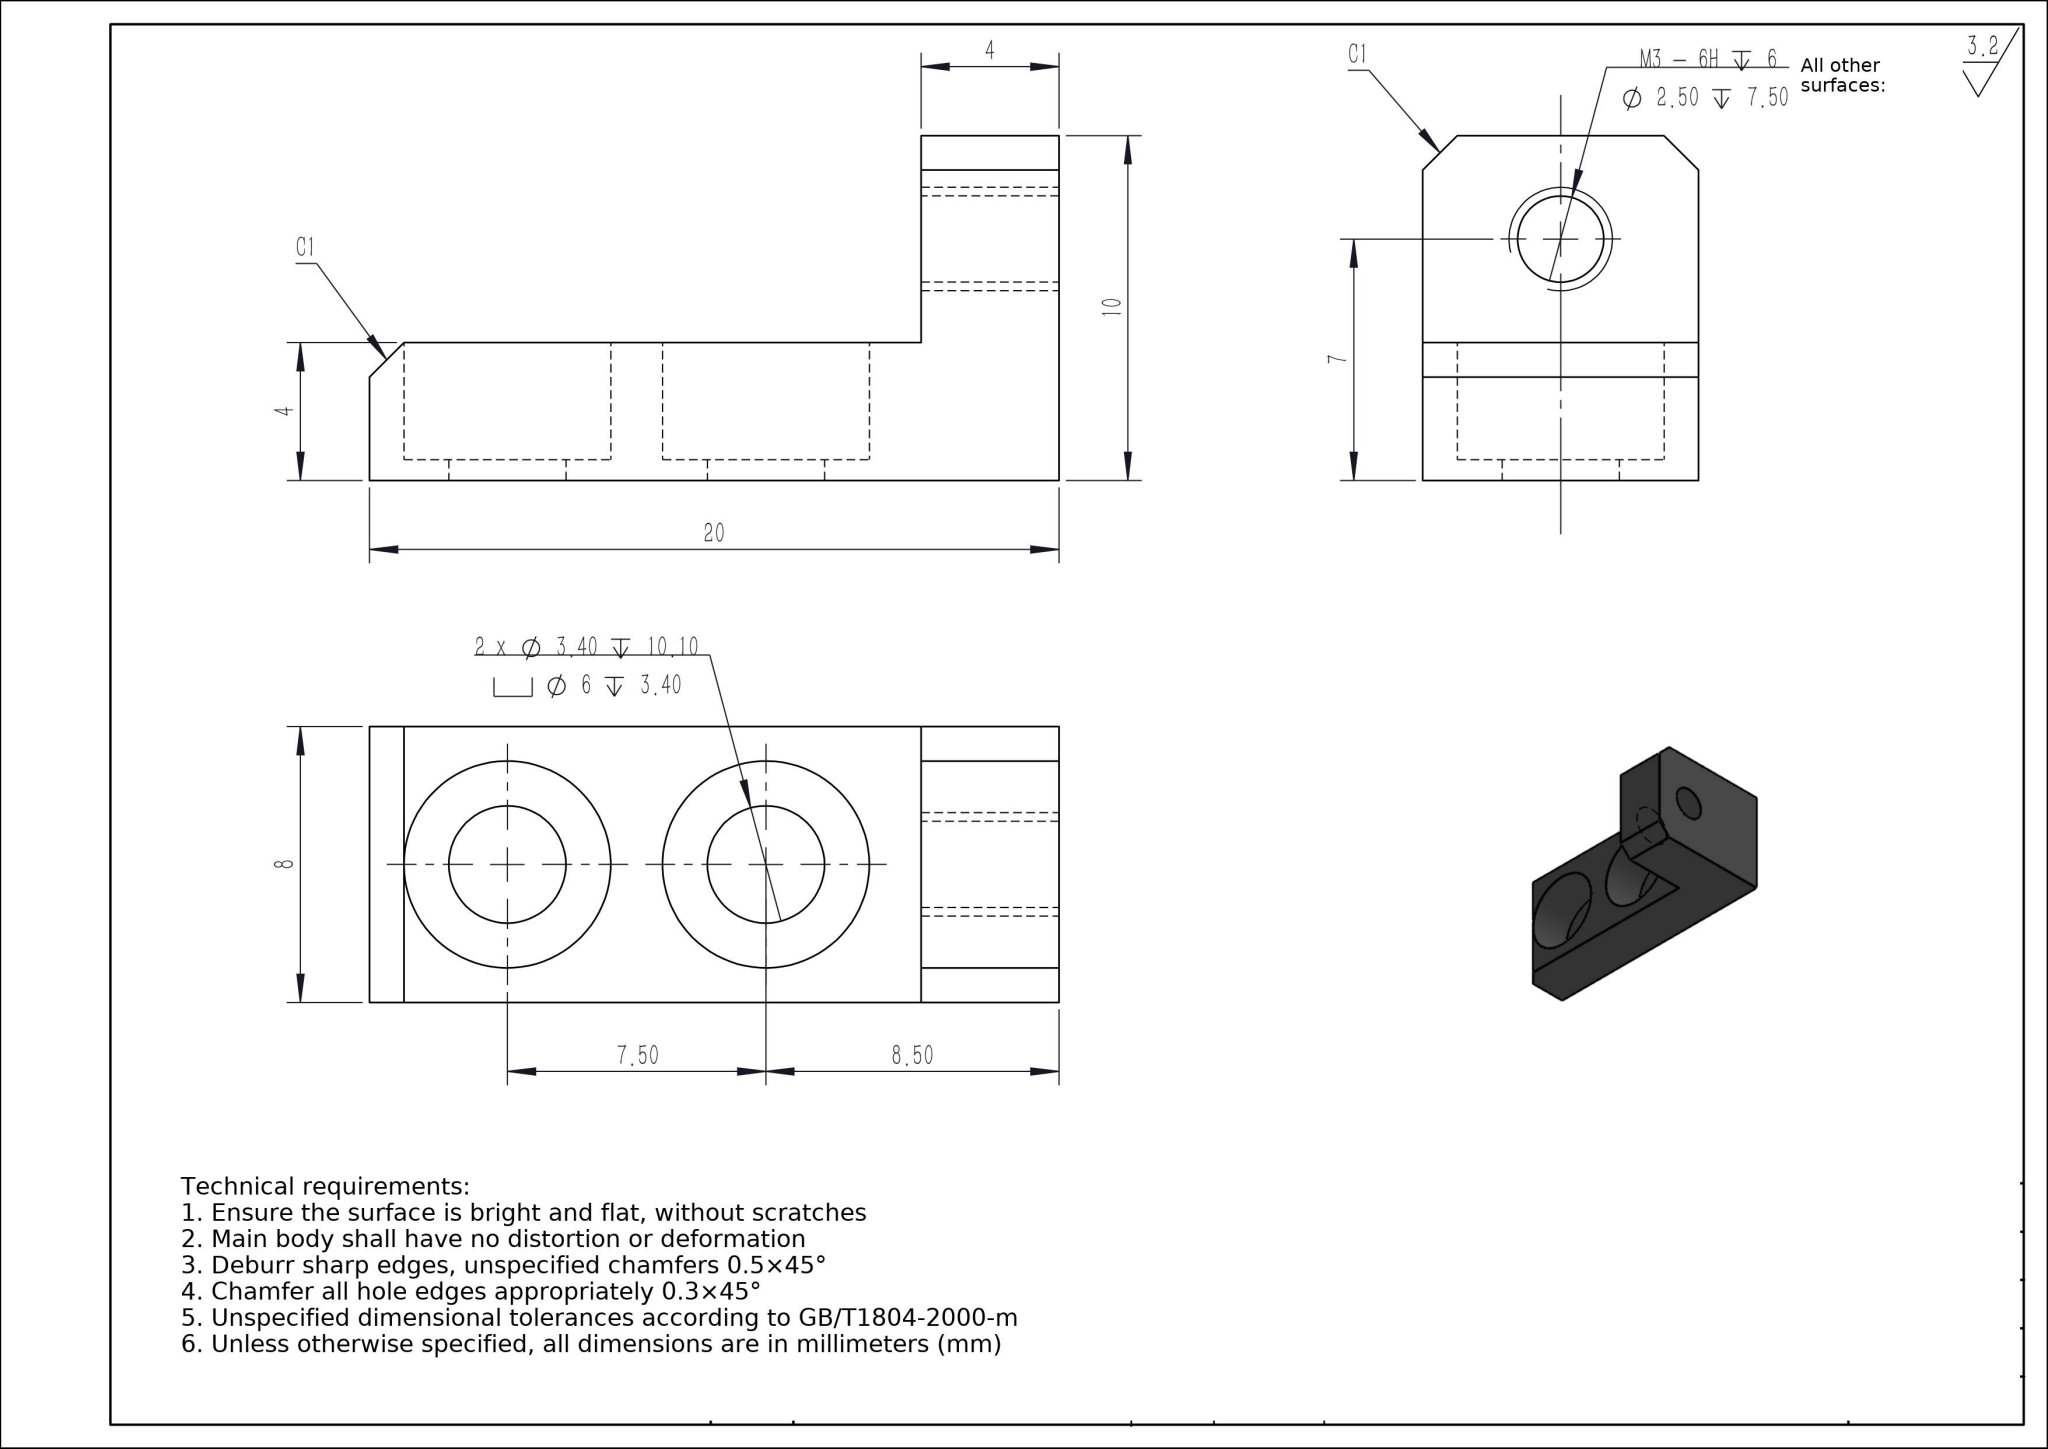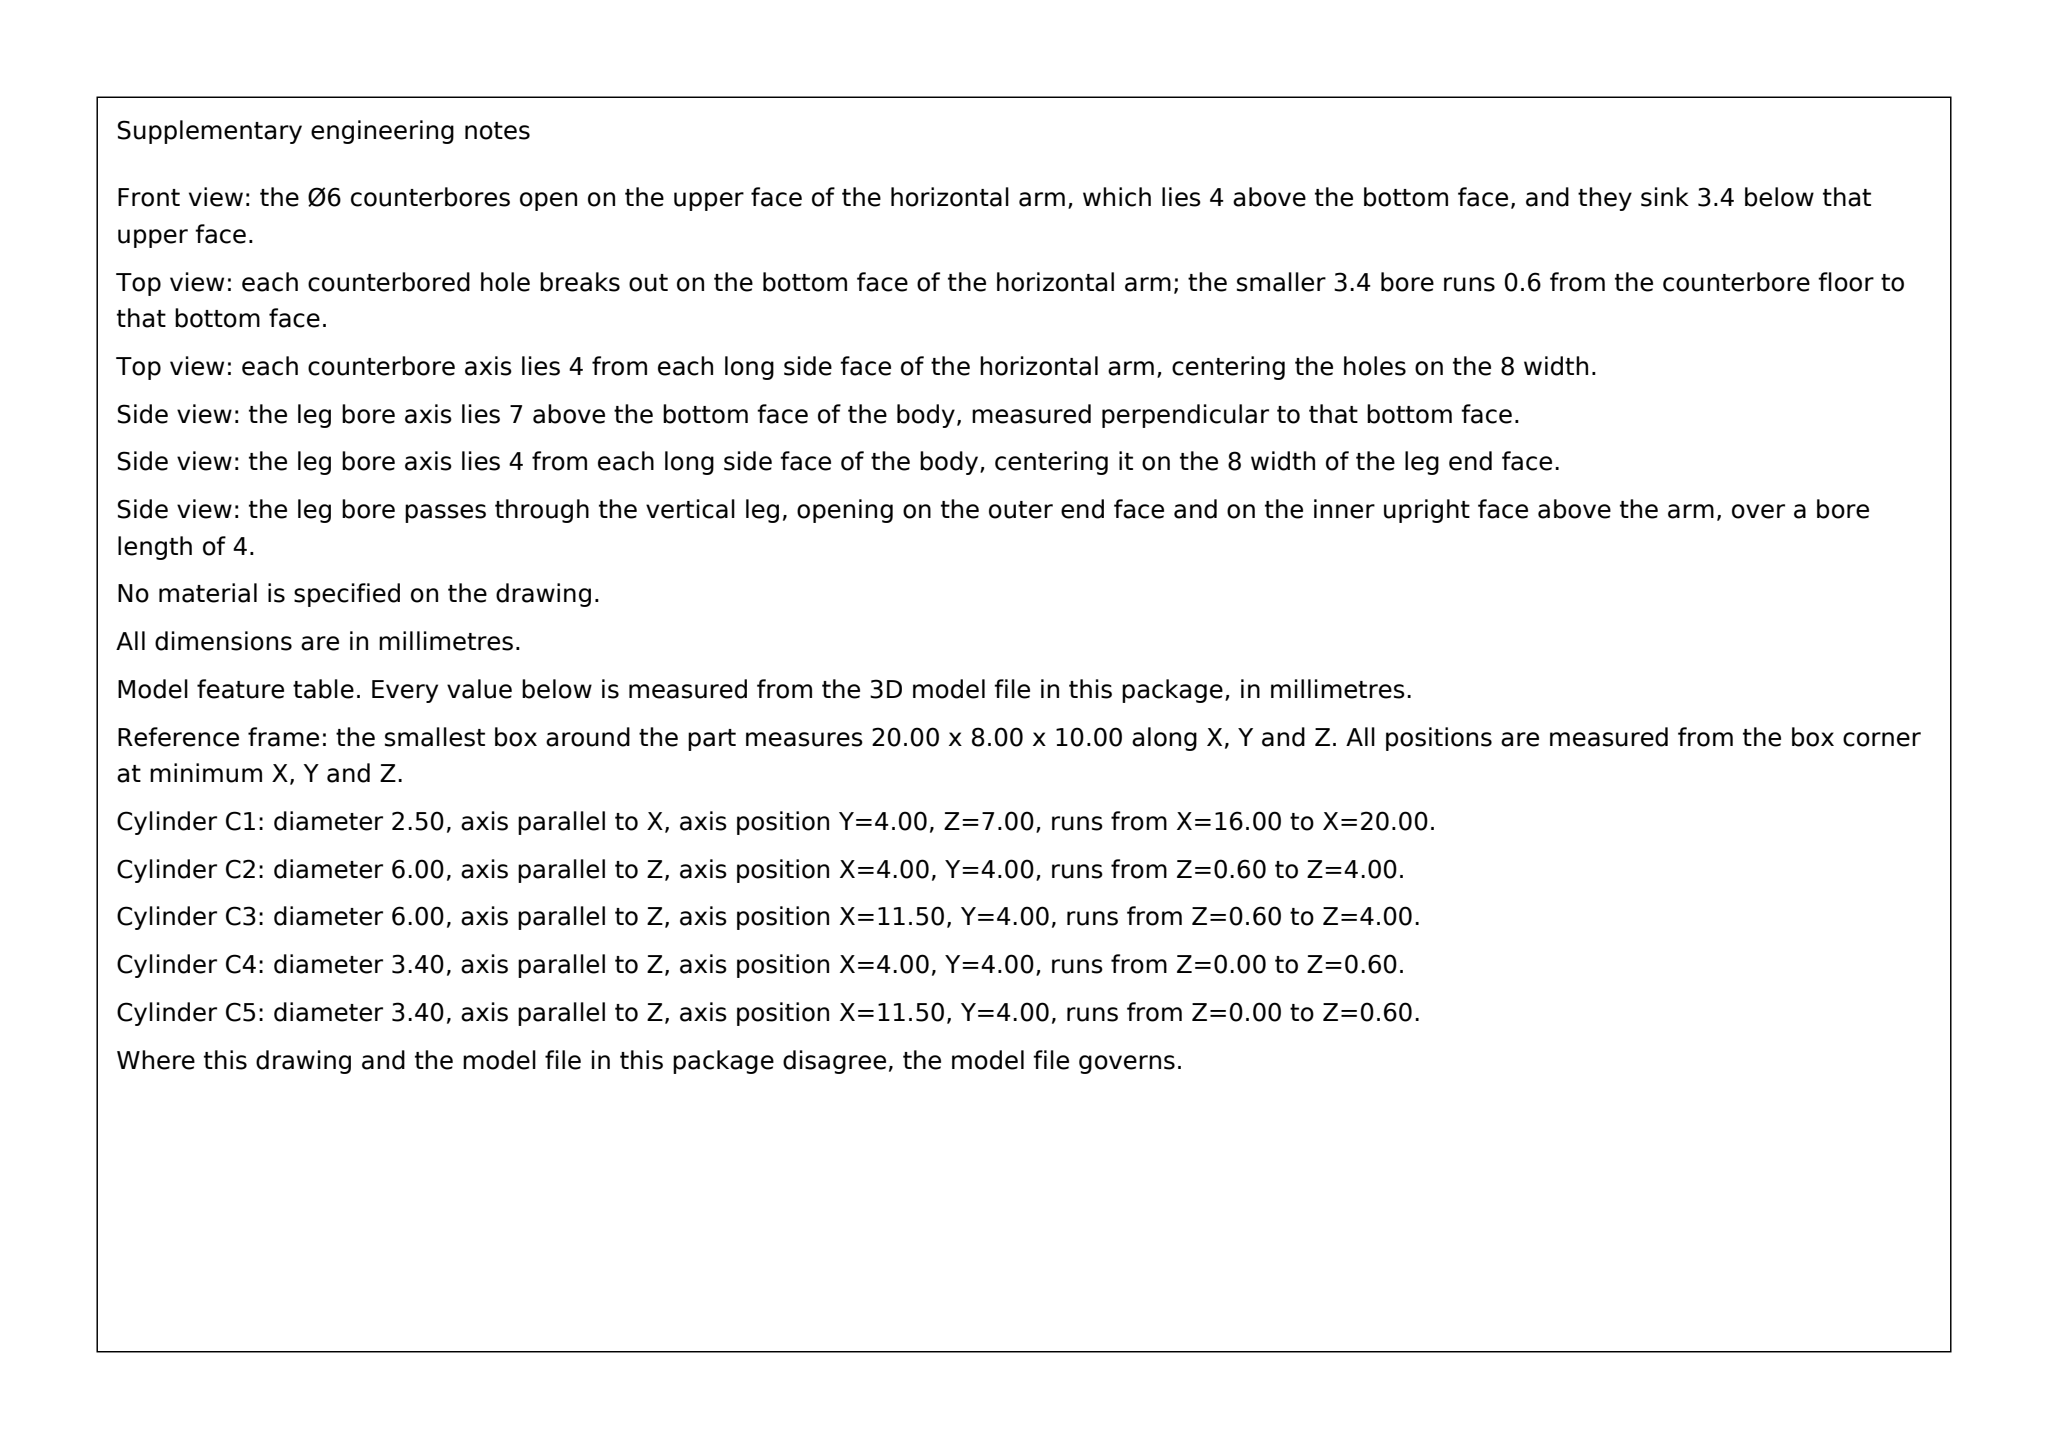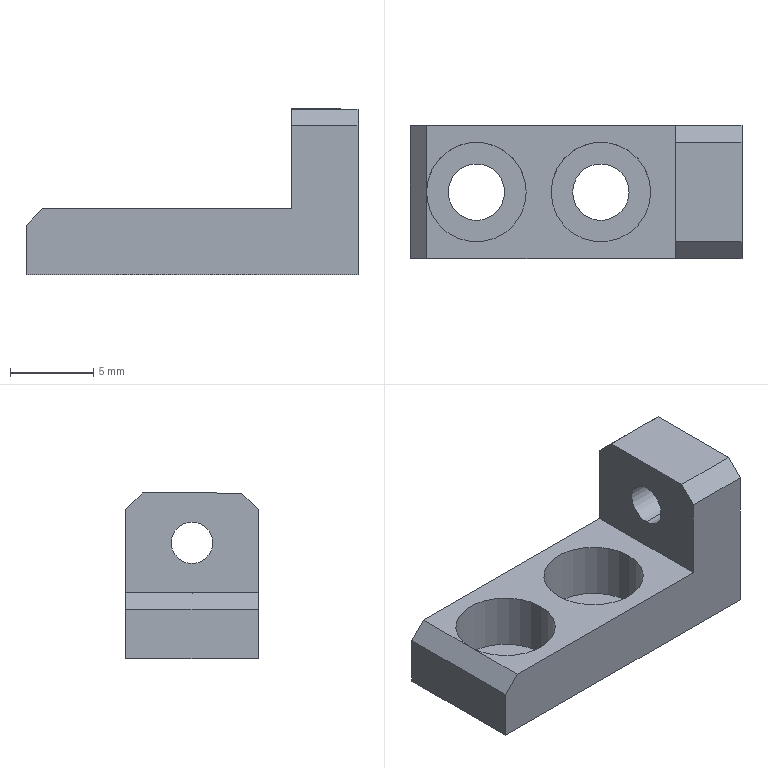Part | SolidWorks | mm | 1 solid | 23 faces | box 20 x 8 x 10 mm | volume 601 mm3 | plane 13 | cylinder 10 | commonest cylinder face diameters 6 x4 3.4 x4 2.5 x2
Drawing notes:
UPRIGHT TOP CORNERS: 2 x C1 (1 x 45 DEG) CHAMFER | from the solid: inclined_planes: two 45 deg faces, size [4,1,1] at bbox_from [16,0,9] and [16,7,9] -> 1x1 chamfer each side of 4 wide upright top edges
STEP:
#1=CARTESIAN_POINT('',(10.,-0.,5.75));
#2=VERTEX_POINT('',#1);
#3=CARTESIAN_POINT('',(10.,-0.,8.25));
#4=VERTEX_POINT('',#3);
#5=CARTESIAN_POINT('',(10.,-0.,7.));
#6=DIRECTION('',(-1.,0.,0.));
#7=DIRECTION('',(0.,0.,1.));
#8=AXIS2_PLACEMENT_3D('',#5,#6,#7);
#9=CIRCLE('',#8,1.25);
#10=EDGE_CURVE('',#2,#4,#9,.T.);
#11=ORIENTED_EDGE('',*,*,#10,.F.);
#12=CARTESIAN_POINT('',(6.,-0.,5.75));
#13=VERTEX_POINT('',#12);
#14=CARTESIAN_POINT('',(6.,-0.,5.75));
#15=DIRECTION('',(-1.,0.,0.));
#16=VECTOR('',#15,1000.);
#17=LINE('',#14,#16);
#18=EDGE_CURVE('',#2,#13,#17,.T.);
#19=ORIENTED_EDGE('',*,*,#18,.T.);
#20=CARTESIAN_POINT('',(6.,-0.,8.25));
#21=VERTEX_POINT('',#20);
#22=CARTESIAN_POINT('',(6.,-0.,7.));
#23=DIRECTION('',(-1.,0.,0.));
#24=DIRECTION('',(0.,0.,1.));
#25=AXIS2_PLACEMENT_3D('',#22,#23,#24);
#26=CIRCLE('',#25,1.25);
#27=EDGE_CURVE('',#13,#21,#26,.T.);
#28=ORIENTED_EDGE('',*,*,#27,.T.);
#29=CARTESIAN_POINT('',(6.,-0.,8.25));
#30=DIRECTION('',(-1.,0.,0.));
#31=VECTOR('',#30,1000.);
#32=LINE('',#29,#31);
#33=EDGE_CURVE('',#4,#21,#32,.T.);
#34=ORIENTED_EDGE('',*,*,#33,.F.);
#35=EDGE_LOOP('',(#11,#19,#28,#34));
#36=FACE_OUTER_BOUND('',#35,.T.);
#37=CARTESIAN_POINT('',(6.,-0.,7.));
#38=DIRECTION('',(-1.,0.,0.));
#39=DIRECTION('',(0.,0.,1.));
#40=AXIS2_PLACEMENT_3D('',#37,#38,#39);
#41=CYLINDRICAL_SURFACE('',#40,1.25);
#42=ADVANCED_FACE('',(#36),#41,.F.);
#43=CARTESIAN_POINT('',(-9.,0.,0.6));
#44=VERTEX_POINT('',#43);
#45=CARTESIAN_POINT('',(-3.,0.,0.6));
#46=VERTEX_POINT('',#45);
#47=CARTESIAN_POINT('',(-6.,0.,0.6));
#48=DIRECTION('',(0.,0.,1.));
#49=DIRECTION('',(1.,0.,0.));
#50=AXIS2_PLACEMENT_3D('',#47,#48,#49);
#51=CIRCLE('',#50,3.);
#52=EDGE_CURVE('',#44,#46,#51,.T.);
#53=ORIENTED_EDGE('',*,*,#52,.F.);
#54=CARTESIAN_POINT('',(-9.,0.,4.));
#55=VERTEX_POINT('',#54);
#56=CARTESIAN_POINT('',(-9.,0.,4.));
#57=DIRECTION('',(0.,0.,1.));
#58=VECTOR('',#57,1000.);
#59=LINE('',#56,#58);
#60=EDGE_CURVE('',#44,#55,#59,.T.);
#61=ORIENTED_EDGE('',*,*,#60,.T.);
#62=CARTESIAN_POINT('',(-3.,0.,4.));
#63=VERTEX_POINT('',#62);
#64=CARTESIAN_POINT('',(-6.,0.,4.));
#65=DIRECTION('',(0.,0.,1.));
#66=DIRECTION('',(1.,0.,0.));
#67=AXIS2_PLACEMENT_3D('',#64,#65,#66);
#68=CIRCLE('',#67,3.);
#69=EDGE_CURVE('',#55,#63,#68,.T.);
#70=ORIENTED_EDGE('',*,*,#69,.T.);
#71=CARTESIAN_POINT('',(-3.,0.,4.));
#72=DIRECTION('',(0.,0.,1.));
#73=VECTOR('',#72,1000.);
#74=LINE('',#71,#73);
#75=EDGE_CURVE('',#46,#63,#74,.T.);
#76=ORIENTED_EDGE('',*,*,#75,.F.);
#77=EDGE_LOOP('',(#53,#61,#70,#76));
#78=FACE_OUTER_BOUND('',#77,.T.);
#79=CARTESIAN_POINT('',(-6.,0.,4.));
#80=DIRECTION('',(0.,0.,1.));
#81=DIRECTION('',(1.,0.,0.));
#82=AXIS2_PLACEMENT_3D('',#79,#80,#81);
#83=CYLINDRICAL_SURFACE('',#82,3.);
#84=ADVANCED_FACE('',(#78),#83,.F.);
#85=CARTESIAN_POINT('',(-7.7,0.,0.));
#86=VERTEX_POINT('',#85);
#87=CARTESIAN_POINT('',(-4.3,0.,0.));
#88=VERTEX_POINT('',#87);
#89=CARTESIAN_POINT('',(-6.,0.,0.));
#90=DIRECTION('',(0.,0.,1.));
#91=DIRECTION('',(1.,0.,0.));
#92=AXIS2_PLACEMENT_3D('',#89,#90,#91);
#93=CIRCLE('',#92,1.7);
#94=EDGE_CURVE('',#86,#88,#93,.T.);
#95=ORIENTED_EDGE('',*,*,#94,.F.);
#96=CARTESIAN_POINT('',(-7.7,0.,0.6));
#97=VERTEX_POINT('',#96);
#98=CARTESIAN_POINT('',(-7.7,0.,4.));
#99=DIRECTION('',(0.,0.,1.));
#100=VECTOR('',#99,1000.);
#101=LINE('',#98,#100);
#102=EDGE_CURVE('',#86,#97,#101,.T.);
#103=ORIENTED_EDGE('',*,*,#102,.T.);
#104=CARTESIAN_POINT('',(-4.3,0.,0.6));
#105=VERTEX_POINT('',#104);
#106=CARTESIAN_POINT('',(-6.,0.,0.6));
#107=DIRECTION('',(0.,0.,1.));
#108=DIRECTION('',(1.,0.,0.));
#109=AXIS2_PLACEMENT_3D('',#106,#107,#108);
#110=CIRCLE('',#109,1.7);
#111=EDGE_CURVE('',#97,#105,#110,.T.);
#112=ORIENTED_EDGE('',*,*,#111,.T.);
#113=CARTESIAN_POINT('',(-4.3,0.,4.));
#114=DIRECTION('',(0.,0.,1.));
#115=VECTOR('',#114,1000.);
#116=LINE('',#113,#115);
#117=EDGE_CURVE('',#88,#105,#116,.T.);
#118=ORIENTED_EDGE('',*,*,#117,.F.);
#119=EDGE_LOOP('',(#95,#103,#112,#118));
#120=FACE_OUTER_BOUND('',#119,.T.);
#121=CARTESIAN_POINT('',(-6.,0.,4.));
#122=DIRECTION('',(0.,0.,1.));
#123=DIRECTION('',(1.,0.,0.));
#124=AXIS2_PLACEMENT_3D('',#121,#122,#123);
#125=CYLINDRICAL_SURFACE('',#124,1.7);
#126=ADVANCED_FACE('',(#120),#125,.F.);
#127=CARTESIAN_POINT('',(-1.5,0.,0.6));
#128=VERTEX_POINT('',#127);
#129=CARTESIAN_POINT('',(4.5,0.,0.6));
#130=VERTEX_POINT('',#129);
#131=CARTESIAN_POINT('',(1.5,0.,0.6));
#132=DIRECTION('',(0.,0.,1.));
#133=DIRECTION('',(1.,0.,0.));
#134=AXIS2_PLACEMENT_3D('',#131,#132,#133);
#135=CIRCLE('',#134,3.);
#136=EDGE_CURVE('',#128,#130,#135,.T.);
#137=ORIENTED_EDGE('',*,*,#136,.F.);
#138=CARTESIAN_POINT('',(-1.5,0.,4.));
#139=VERTEX_POINT('',#138);
#140=CARTESIAN_POINT('',(-1.5,0.,4.));
#141=DIRECTION('',(0.,0.,1.));
#142=VECTOR('',#141,1000.);
#143=LINE('',#140,#142);
#144=EDGE_CURVE('',#128,#139,#143,.T.);
#145=ORIENTED_EDGE('',*,*,#144,.T.);
#146=CARTESIAN_POINT('',(4.5,0.,4.));
#147=VERTEX_POINT('',#146);
#148=CARTESIAN_POINT('',(1.5,0.,4.));
#149=DIRECTION('',(0.,0.,1.));
#150=DIRECTION('',(1.,0.,0.));
#151=AXIS2_PLACEMENT_3D('',#148,#149,#150);
#152=CIRCLE('',#151,3.);
#153=EDGE_CURVE('',#139,#147,#152,.T.);
#154=ORIENTED_EDGE('',*,*,#153,.T.);
#155=CARTESIAN_POINT('',(4.5,0.,4.));
#156=DIRECTION('',(0.,0.,1.));
#157=VECTOR('',#156,1000.);
#158=LINE('',#155,#157);
#159=EDGE_CURVE('',#130,#147,#158,.T.);
#160=ORIENTED_EDGE('',*,*,#159,.F.);
#161=EDGE_LOOP('',(#137,#145,#154,#160));
#162=FACE_OUTER_BOUND('',#161,.T.);
#163=CARTESIAN_POINT('',(1.5,0.,4.));
#164=DIRECTION('',(0.,0.,1.));
#165=DIRECTION('',(1.,0.,0.));
#166=AXIS2_PLACEMENT_3D('',#163,#164,#165);
#167=CYLINDRICAL_SURFACE('',#166,3.);
#168=ADVANCED_FACE('',(#162),#167,.F.);
#169=CARTESIAN_POINT('',(-0.2,0.,0.));
#170=VERTEX_POINT('',#169);
#171=CARTESIAN_POINT('',(3.2,0.,0.));
#172=VERTEX_POINT('',#171);
#173=CARTESIAN_POINT('',(1.5,0.,0.));
#174=DIRECTION('',(0.,0.,1.));
#175=DIRECTION('',(1.,0.,0.));
#176=AXIS2_PLACEMENT_3D('',#173,#174,#175);
#177=CIRCLE('',#176,1.7);
#178=EDGE_CURVE('',#170,#172,#177,.T.);
#179=ORIENTED_EDGE('',*,*,#178,.F.);
#180=CARTESIAN_POINT('',(-0.2,0.,0.6));
#181=VERTEX_POINT('',#180);
#182=CARTESIAN_POINT('',(-0.2,0.,4.));
#183=DIRECTION('',(0.,0.,1.));
#184=VECTOR('',#183,1000.);
#185=LINE('',#182,#184);
#186=EDGE_CURVE('',#170,#181,#185,.T.);
#187=ORIENTED_EDGE('',*,*,#186,.T.);
#188=CARTESIAN_POINT('',(3.2,0.,0.6));
#189=VERTEX_POINT('',#188);
#190=CARTESIAN_POINT('',(1.5,0.,0.6));
#191=DIRECTION('',(0.,0.,1.));
#192=DIRECTION('',(1.,0.,0.));
#193=AXIS2_PLACEMENT_3D('',#190,#191,#192);
#194=CIRCLE('',#193,1.7);
#195=EDGE_CURVE('',#181,#189,#194,.T.);
#196=ORIENTED_EDGE('',*,*,#195,.T.);
#197=CARTESIAN_POINT('',(3.2,0.,4.));
#198=DIRECTION('',(0.,0.,1.));
#199=VECTOR('',#198,1000.);
#200=LINE('',#197,#199);
#201=EDGE_CURVE('',#172,#189,#200,.T.);
#202=ORIENTED_EDGE('',*,*,#201,.F.);
#203=EDGE_LOOP('',(#179,#187,#196,#202));
#204=FACE_OUTER_BOUND('',#203,.T.);
#205=CARTESIAN_POINT('',(1.5,0.,4.));
#206=DIRECTION('',(0.,0.,1.));
#207=DIRECTION('',(1.,0.,0.));
#208=AXIS2_PLACEMENT_3D('',#205,#206,#207);
#209=CYLINDRICAL_SURFACE('',#208,1.7);
#210=ADVANCED_FACE('',(#204),#209,.F.);
#211=CARTESIAN_POINT('',(-10.,-4.,3.));
#212=VERTEX_POINT('',#211);
#213=CARTESIAN_POINT('',(-10.,-4.,0.));
#214=VERTEX_POINT('',#213);
#215=CARTESIAN_POINT('',(-10.,-4.,4.));
#216=DIRECTION('',(0.,0.,-1.));
#217=VECTOR('',#216,1000.);
#218=LINE('',#215,#217);
#219=EDGE_CURVE('',#212,#214,#218,.T.);
#220=ORIENTED_EDGE('',*,*,#219,.F.);
#221=CARTESIAN_POINT('',(-10.,4.,3.));
#222=VERTEX_POINT('',#221);
#223=CARTESIAN_POINT('',(-10.,4.,3.));
#224=DIRECTION('',(0.,1.,0.));
#225=VECTOR('',#224,1000.);
#226=LINE('',#223,#225);
#227=EDGE_CURVE('',#212,#222,#226,.T.);
#228=ORIENTED_EDGE('',*,*,#227,.T.);
#229=CARTESIAN_POINT('',(-10.,4.,0.));
#230=VERTEX_POINT('',#229);
#231=CARTESIAN_POINT('',(-10.,4.,4.));
#232=DIRECTION('',(0.,0.,-1.));
#233=VECTOR('',#232,1000.);
#234=LINE('',#231,#233);
#235=EDGE_CURVE('',#222,#230,#234,.T.);
#236=ORIENTED_EDGE('',*,*,#235,.T.);
#237=CARTESIAN_POINT('',(-10.,-4.,0.));
#238=DIRECTION('',(0.,-1.,0.));
#239=VECTOR('',#238,1000.);
#240=LINE('',#237,#239);
#241=EDGE_CURVE('',#230,#214,#240,.T.);
#242=ORIENTED_EDGE('',*,*,#241,.T.);
#243=EDGE_LOOP('',(#220,#228,#236,#242));
#244=FACE_OUTER_BOUND('',#243,.T.);
#245=CARTESIAN_POINT('',(-10.,-4.,4.));
#246=DIRECTION('',(1.,0.,0.));
#247=DIRECTION('',(0.,0.,-1.));
#248=AXIS2_PLACEMENT_3D('',#245,#246,#247);
#249=PLANE('',#248);
#250=ADVANCED_FACE('',(#244),#249,.F.);
#251=CARTESIAN_POINT('',(10.,-4.,9.));
#252=VERTEX_POINT('',#251);
#253=CARTESIAN_POINT('',(10.,-4.,0.));
#254=VERTEX_POINT('',#253);
#255=CARTESIAN_POINT('',(10.,-4.,4.));
#256=DIRECTION('',(0.,0.,-1.));
#257=VECTOR('',#256,1000.);
#258=LINE('',#255,#257);
#259=EDGE_CURVE('',#252,#254,#258,.T.);
#260=ORIENTED_EDGE('',*,*,#259,.F.);
#261=CARTESIAN_POINT('',(6.,-4.,9.));
#262=VERTEX_POINT('',#261);
#263=CARTESIAN_POINT('',(6.,-4.,9.));
#264=DIRECTION('',(-1.,-0.,0.));
#265=VECTOR('',#264,1000.);
#266=LINE('',#263,#265);
#267=EDGE_CURVE('',#252,#262,#266,.T.);
#268=ORIENTED_EDGE('',*,*,#267,.T.);
#269=CARTESIAN_POINT('',(6.,-4.,4.));
#270=VERTEX_POINT('',#269);
#271=CARTESIAN_POINT('',(6.,-4.,10.));
#272=DIRECTION('',(0.,0.,-1.));
#273=VECTOR('',#272,1000.);
#274=LINE('',#271,#273);
#275=EDGE_CURVE('',#262,#270,#274,.T.);
#276=ORIENTED_EDGE('',*,*,#275,.T.);
#277=CARTESIAN_POINT('',(-9.,-4.,4.));
#278=VERTEX_POINT('',#277);
#279=CARTESIAN_POINT('',(10.,-4.,4.));
#280=DIRECTION('',(1.,0.,0.));
#281=VECTOR('',#280,1000.);
#282=LINE('',#279,#281);
#283=EDGE_CURVE('',#278,#270,#282,.T.);
#284=ORIENTED_EDGE('',*,*,#283,.F.);
#285=CARTESIAN_POINT('',(-9.,-4.,4.));
#286=DIRECTION('',(-0.7071,-0.,-0.7071));
#287=VECTOR('',#286,1000.);
#288=LINE('',#285,#287);
#289=EDGE_CURVE('',#278,#212,#288,.T.);
#290=ORIENTED_EDGE('',*,*,#289,.T.);
#291=ORIENTED_EDGE('',*,*,#219,.T.);
#292=CARTESIAN_POINT('',(10.,-4.,0.));
#293=DIRECTION('',(1.,0.,0.));
#294=VECTOR('',#293,1000.);
#295=LINE('',#292,#294);
#296=EDGE_CURVE('',#214,#254,#295,.T.);
#297=ORIENTED_EDGE('',*,*,#296,.T.);
#298=EDGE_LOOP('',(#260,#268,#276,#284,#290,#291,#297));
#299=FACE_OUTER_BOUND('',#298,.T.);
#300=CARTESIAN_POINT('',(10.,-4.,4.));
#301=DIRECTION('',(-0.,1.,0.));
#302=DIRECTION('',(-1.,-0.,0.));
#303=AXIS2_PLACEMENT_3D('',#300,#301,#302);
#304=PLANE('',#303);
#305=ADVANCED_FACE('',(#299),#304,.F.);
#306=CARTESIAN_POINT('',(10.,-0.,7.));
#307=DIRECTION('',(-1.,0.,0.));
#308=DIRECTION('',(0.,0.,1.));
#309=AXIS2_PLACEMENT_3D('',#306,#307,#308);
#310=CIRCLE('',#309,1.25);
#311=EDGE_CURVE('',#4,#2,#310,.T.);
#312=ORIENTED_EDGE('',*,*,#311,.T.);
#313=ORIENTED_EDGE('',*,*,#10,.T.);
#314=EDGE_LOOP('',(#312,#313));
#315=FACE_BOUND('',#314,.T.);
#316=CARTESIAN_POINT('',(10.,4.,9.));
#317=VERTEX_POINT('',#316);
#318=CARTESIAN_POINT('',(10.,4.,0.));
#319=VERTEX_POINT('',#318);
#320=CARTESIAN_POINT('',(10.,4.,4.));
#321=DIRECTION('',(0.,0.,-1.));
#322=VECTOR('',#321,1000.);
#323=LINE('',#320,#322);
#324=EDGE_CURVE('',#317,#319,#323,.T.);
#325=ORIENTED_EDGE('',*,*,#324,.F.);
#326=CARTESIAN_POINT('',(10.,3.,10.));
#327=VERTEX_POINT('',#326);
#328=CARTESIAN_POINT('',(10.,3.,10.));
#329=DIRECTION('',(0.,-0.7071,0.7071));
#330=VECTOR('',#329,1000.);
#331=LINE('',#328,#330);
#332=EDGE_CURVE('',#317,#327,#331,.T.);
#333=ORIENTED_EDGE('',*,*,#332,.T.);
#334=CARTESIAN_POINT('',(10.,-3.,10.));
#335=VERTEX_POINT('',#334);
#336=CARTESIAN_POINT('',(10.,-4.,10.));
#337=DIRECTION('',(0.,1.,0.));
#338=VECTOR('',#337,1000.);
#339=LINE('',#336,#338);
#340=EDGE_CURVE('',#335,#327,#339,.T.);
#341=ORIENTED_EDGE('',*,*,#340,.F.);
#342=CARTESIAN_POINT('',(10.,-3.,10.));
#343=DIRECTION('',(0.,-0.7071,-0.7071));
#344=VECTOR('',#343,1000.);
#345=LINE('',#342,#344);
#346=EDGE_CURVE('',#335,#252,#345,.T.);
#347=ORIENTED_EDGE('',*,*,#346,.T.);
#348=ORIENTED_EDGE('',*,*,#259,.T.);
#349=CARTESIAN_POINT('',(10.,-4.,0.));
#350=DIRECTION('',(0.,1.,0.));
#351=VECTOR('',#350,1000.);
#352=LINE('',#349,#351);
#353=EDGE_CURVE('',#254,#319,#352,.T.);
#354=ORIENTED_EDGE('',*,*,#353,.T.);
#355=EDGE_LOOP('',(#325,#333,#341,#347,#348,#354));
#356=FACE_OUTER_BOUND('',#355,.T.);
#357=CARTESIAN_POINT('',(10.,-4.,4.));
#358=DIRECTION('',(-1.,0.,0.));
#359=DIRECTION('',(0.,0.,1.));
#360=AXIS2_PLACEMENT_3D('',#357,#358,#359);
#361=PLANE('',#360);
#362=ADVANCED_FACE('',(#315,#356),#361,.F.);
#363=CARTESIAN_POINT('',(6.,4.,9.));
#364=VERTEX_POINT('',#363);
#365=CARTESIAN_POINT('',(6.,4.,4.));
#366=VERTEX_POINT('',#365);
#367=CARTESIAN_POINT('',(6.,4.,10.));
#368=DIRECTION('',(0.,0.,-1.));
#369=VECTOR('',#368,1000.);
#370=LINE('',#367,#369);
#371=EDGE_CURVE('',#364,#366,#370,.T.);
#372=ORIENTED_EDGE('',*,*,#371,.F.);
#373=CARTESIAN_POINT('',(10.,4.,9.));
#374=DIRECTION('',(1.,0.,0.));
#375=VECTOR('',#374,1000.);
#376=LINE('',#373,#375);
#377=EDGE_CURVE('',#364,#317,#376,.T.);
#378=ORIENTED_EDGE('',*,*,#377,.T.);
#379=ORIENTED_EDGE('',*,*,#324,.T.);
#380=CARTESIAN_POINT('',(10.,4.,0.));
#381=DIRECTION('',(-1.,-0.,0.));
#382=VECTOR('',#381,1000.);
#383=LINE('',#380,#382);
#384=EDGE_CURVE('',#319,#230,#383,.T.);
#385=ORIENTED_EDGE('',*,*,#384,.T.);
#386=ORIENTED_EDGE('',*,*,#235,.F.);
#387=CARTESIAN_POINT('',(-9.,4.,4.));
#388=VERTEX_POINT('',#387);
#389=CARTESIAN_POINT('',(-9.,4.,4.));
#390=DIRECTION('',(0.7071,0.,0.7071));
#391=VECTOR('',#390,1000.);
#392=LINE('',#389,#391);
#393=EDGE_CURVE('',#222,#388,#392,.T.);
#394=ORIENTED_EDGE('',*,*,#393,.T.);
#395=CARTESIAN_POINT('',(10.,4.,4.));
#396=DIRECTION('',(-1.,-0.,0.));
#397=VECTOR('',#396,1000.);
#398=LINE('',#395,#397);
#399=EDGE_CURVE('',#366,#388,#398,.T.);
#400=ORIENTED_EDGE('',*,*,#399,.F.);
#401=EDGE_LOOP('',(#372,#378,#379,#385,#386,#394,#400));
#402=FACE_OUTER_BOUND('',#401,.T.);
#403=CARTESIAN_POINT('',(10.,4.,4.));
#404=DIRECTION('',(0.,-1.,0.));
#405=DIRECTION('',(1.,0.,0.));
#406=AXIS2_PLACEMENT_3D('',#403,#404,#405);
#407=PLANE('',#406);
#408=ADVANCED_FACE('',(#402),#407,.F.);
#409=CARTESIAN_POINT('',(6.,-4.,4.));
#410=DIRECTION('',(0.,-1.,0.));
#411=VECTOR('',#410,1000.);
#412=LINE('',#409,#411);
#413=EDGE_CURVE('',#366,#270,#412,.T.);
#414=ORIENTED_EDGE('',*,*,#413,.F.);
#415=ORIENTED_EDGE('',*,*,#399,.T.);
#416=CARTESIAN_POINT('',(-9.,-4.,4.));
#417=DIRECTION('',(0.,-1.,0.));
#418=VECTOR('',#417,1000.);
#419=LINE('',#416,#418);
#420=EDGE_CURVE('',#388,#55,#419,.T.);
#421=ORIENTED_EDGE('',*,*,#420,.T.);
#422=CARTESIAN_POINT('',(-6.,0.,4.));
#423=DIRECTION('',(0.,0.,1.));
#424=DIRECTION('',(1.,0.,0.));
#425=AXIS2_PLACEMENT_3D('',#422,#423,#424);
#426=CIRCLE('',#425,3.);
#427=EDGE_CURVE('',#63,#55,#426,.T.);
#428=ORIENTED_EDGE('',*,*,#427,.F.);
#429=ORIENTED_EDGE('',*,*,#69,.F.);
#430=CARTESIAN_POINT('',(-9.,-4.,4.));
#431=DIRECTION('',(0.,-1.,0.));
#432=VECTOR('',#431,1000.);
#433=LINE('',#430,#432);
#434=EDGE_CURVE('',#55,#278,#433,.T.);
#435=ORIENTED_EDGE('',*,*,#434,.T.);
#436=ORIENTED_EDGE('',*,*,#283,.T.);
#437=EDGE_LOOP('',(#414,#415,#421,#428,#429,#435,#436));
#438=FACE_OUTER_BOUND('',#437,.T.);
#439=CARTESIAN_POINT('',(1.5,0.,4.));
#440=DIRECTION('',(0.,0.,1.));
#441=DIRECTION('',(1.,0.,0.));
#442=AXIS2_PLACEMENT_3D('',#439,#440,#441);
#443=CIRCLE('',#442,3.);
#444=EDGE_CURVE('',#147,#139,#443,.T.);
#445=ORIENTED_EDGE('',*,*,#444,.F.);
#446=ORIENTED_EDGE('',*,*,#153,.F.);
#447=EDGE_LOOP('',(#445,#446));
#448=FACE_BOUND('',#447,.T.);
#449=CARTESIAN_POINT('',(0.,0.,4.));
#450=DIRECTION('',(0.,0.,1.));
#451=DIRECTION('',(1.,0.,0.));
#452=AXIS2_PLACEMENT_3D('',#449,#450,#451);
#453=PLANE('',#452);
#454=ADVANCED_FACE('',(#438,#448),#453,.T.);
#455=CARTESIAN_POINT('',(-6.,0.,0.));
#456=DIRECTION('',(0.,0.,1.));
#457=DIRECTION('',(1.,0.,0.));
#458=AXIS2_PLACEMENT_3D('',#455,#456,#457);
#459=CIRCLE('',#458,1.7);
#460=EDGE_CURVE('',#88,#86,#459,.T.);
#461=ORIENTED_EDGE('',*,*,#460,.T.);
#462=ORIENTED_EDGE('',*,*,#94,.T.);
#463=EDGE_LOOP('',(#461,#462));
#464=FACE_BOUND('',#463,.T.);
#465=CARTESIAN_POINT('',(1.5,0.,0.));
#466=DIRECTION('',(0.,0.,1.));
#467=DIRECTION('',(1.,0.,0.));
#468=AXIS2_PLACEMENT_3D('',#465,#466,#467);
#469=CIRCLE('',#468,1.7);
#470=EDGE_CURVE('',#172,#170,#469,.T.);
#471=ORIENTED_EDGE('',*,*,#470,.T.);
#472=ORIENTED_EDGE('',*,*,#178,.T.);
#473=EDGE_LOOP('',(#471,#472));
#474=FACE_BOUND('',#473,.T.);
#475=ORIENTED_EDGE('',*,*,#241,.F.);
#476=ORIENTED_EDGE('',*,*,#384,.F.);
#477=ORIENTED_EDGE('',*,*,#353,.F.);
#478=ORIENTED_EDGE('',*,*,#296,.F.);
#479=EDGE_LOOP('',(#475,#476,#477,#478));
#480=FACE_OUTER_BOUND('',#479,.T.);
#481=CARTESIAN_POINT('',(0.,0.,0.));
#482=DIRECTION('',(0.,0.,1.));
#483=DIRECTION('',(1.,0.,0.));
#484=AXIS2_PLACEMENT_3D('',#481,#482,#483);
#485=PLANE('',#484);
#486=ADVANCED_FACE('',(#464,#474,#480),#485,.F.);
#487=ORIENTED_EDGE('',*,*,#186,.F.);
#488=ORIENTED_EDGE('',*,*,#470,.F.);
#489=ORIENTED_EDGE('',*,*,#201,.T.);
#490=CARTESIAN_POINT('',(1.5,0.,0.6));
#491=DIRECTION('',(0.,0.,1.));
#492=DIRECTION('',(1.,0.,0.));
#493=AXIS2_PLACEMENT_3D('',#490,#491,#492);
#494=CIRCLE('',#493,1.7);
#495=EDGE_CURVE('',#189,#181,#494,.T.);
#496=ORIENTED_EDGE('',*,*,#495,.T.);
#497=EDGE_LOOP('',(#487,#488,#489,#496));
#498=FACE_OUTER_BOUND('',#497,.T.);
#499=CARTESIAN_POINT('',(1.5,0.,4.));
#500=DIRECTION('',(0.,0.,1.));
#501=DIRECTION('',(1.,0.,0.));
#502=AXIS2_PLACEMENT_3D('',#499,#500,#501);
#503=CYLINDRICAL_SURFACE('',#502,1.7);
#504=ADVANCED_FACE('',(#498),#503,.F.);
#505=ORIENTED_EDGE('',*,*,#495,.F.);
#506=ORIENTED_EDGE('',*,*,#195,.F.);
#507=EDGE_LOOP('',(#505,#506));
#508=FACE_BOUND('',#507,.T.);
#509=CARTESIAN_POINT('',(1.5,0.,0.6));
#510=DIRECTION('',(0.,0.,1.));
#511=DIRECTION('',(1.,0.,0.));
#512=AXIS2_PLACEMENT_3D('',#509,#510,#511);
#513=CIRCLE('',#512,3.);
#514=EDGE_CURVE('',#130,#128,#513,.T.);
#515=ORIENTED_EDGE('',*,*,#514,.T.);
#516=ORIENTED_EDGE('',*,*,#136,.T.);
#517=EDGE_LOOP('',(#515,#516));
#518=FACE_OUTER_BOUND('',#517,.T.);
#519=CARTESIAN_POINT('',(3.2,0.,0.6));
#520=DIRECTION('',(0.,0.,-1.));
#521=DIRECTION('',(-1.,0.,0.));
#522=AXIS2_PLACEMENT_3D('',#519,#520,#521);
#523=PLANE('',#522);
#524=ADVANCED_FACE('',(#508,#518),#523,.F.);
#525=ORIENTED_EDGE('',*,*,#144,.F.);
#526=ORIENTED_EDGE('',*,*,#514,.F.);
#527=ORIENTED_EDGE('',*,*,#159,.T.);
#528=ORIENTED_EDGE('',*,*,#444,.T.);
#529=EDGE_LOOP('',(#525,#526,#527,#528));
#530=FACE_OUTER_BOUND('',#529,.T.);
#531=CARTESIAN_POINT('',(1.5,0.,4.));
#532=DIRECTION('',(0.,0.,1.));
#533=DIRECTION('',(1.,0.,0.));
#534=AXIS2_PLACEMENT_3D('',#531,#532,#533);
#535=CYLINDRICAL_SURFACE('',#534,3.);
#536=ADVANCED_FACE('',(#530),#535,.F.);
#537=ORIENTED_EDGE('',*,*,#102,.F.);
#538=ORIENTED_EDGE('',*,*,#460,.F.);
#539=ORIENTED_EDGE('',*,*,#117,.T.);
#540=CARTESIAN_POINT('',(-6.,0.,0.6));
#541=DIRECTION('',(0.,0.,1.));
#542=DIRECTION('',(1.,0.,0.));
#543=AXIS2_PLACEMENT_3D('',#540,#541,#542);
#544=CIRCLE('',#543,1.7);
#545=EDGE_CURVE('',#105,#97,#544,.T.);
#546=ORIENTED_EDGE('',*,*,#545,.T.);
#547=EDGE_LOOP('',(#537,#538,#539,#546));
#548=FACE_OUTER_BOUND('',#547,.T.);
#549=CARTESIAN_POINT('',(-6.,0.,4.));
#550=DIRECTION('',(0.,0.,1.));
#551=DIRECTION('',(1.,0.,0.));
#552=AXIS2_PLACEMENT_3D('',#549,#550,#551);
#553=CYLINDRICAL_SURFACE('',#552,1.7);
#554=ADVANCED_FACE('',(#548),#553,.F.);
#555=ORIENTED_EDGE('',*,*,#545,.F.);
#556=ORIENTED_EDGE('',*,*,#111,.F.);
#557=EDGE_LOOP('',(#555,#556));
#558=FACE_BOUND('',#557,.T.);
#559=CARTESIAN_POINT('',(-6.,0.,0.6));
#560=DIRECTION('',(0.,0.,1.));
#561=DIRECTION('',(1.,0.,0.));
#562=AXIS2_PLACEMENT_3D('',#559,#560,#561);
#563=CIRCLE('',#562,3.);
#564=EDGE_CURVE('',#46,#44,#563,.T.);
#565=ORIENTED_EDGE('',*,*,#564,.T.);
#566=ORIENTED_EDGE('',*,*,#52,.T.);
#567=EDGE_LOOP('',(#565,#566));
#568=FACE_OUTER_BOUND('',#567,.T.);
#569=CARTESIAN_POINT('',(-4.3,0.,0.6));
#570=DIRECTION('',(0.,0.,-1.));
#571=DIRECTION('',(-1.,0.,0.));
#572=AXIS2_PLACEMENT_3D('',#569,#570,#571);
#573=PLANE('',#572);
#574=ADVANCED_FACE('',(#558,#568),#573,.F.);
#575=ORIENTED_EDGE('',*,*,#60,.F.);
#576=ORIENTED_EDGE('',*,*,#564,.F.);
#577=ORIENTED_EDGE('',*,*,#75,.T.);
#578=ORIENTED_EDGE('',*,*,#427,.T.);
#579=EDGE_LOOP('',(#575,#576,#577,#578));
#580=FACE_OUTER_BOUND('',#579,.T.);
#581=CARTESIAN_POINT('',(-6.,0.,4.));
#582=DIRECTION('',(0.,0.,1.));
#583=DIRECTION('',(1.,0.,0.));
#584=AXIS2_PLACEMENT_3D('',#581,#582,#583);
#585=CYLINDRICAL_SURFACE('',#584,3.);
#586=ADVANCED_FACE('',(#580),#585,.F.);
#587=ORIENTED_EDGE('',*,*,#393,.F.);
#588=ORIENTED_EDGE('',*,*,#227,.F.);
#589=ORIENTED_EDGE('',*,*,#289,.F.);
#590=ORIENTED_EDGE('',*,*,#434,.F.);
#591=ORIENTED_EDGE('',*,*,#420,.F.);
#592=EDGE_LOOP('',(#587,#588,#589,#590,#591));
#593=FACE_OUTER_BOUND('',#592,.T.);
#594=CARTESIAN_POINT('',(-9.,0.,4.));
#595=DIRECTION('',(-0.7071,0.,0.7071));
#596=DIRECTION('',(0.,1.,0.));
#597=AXIS2_PLACEMENT_3D('',#594,#595,#596);
#598=PLANE('',#597);
#599=ADVANCED_FACE('',(#593),#598,.T.);
#600=CARTESIAN_POINT('',(6.,-0.,7.));
#601=DIRECTION('',(-1.,0.,0.));
#602=DIRECTION('',(0.,0.,1.));
#603=AXIS2_PLACEMENT_3D('',#600,#601,#602);
#604=CIRCLE('',#603,1.25);
#605=EDGE_CURVE('',#21,#13,#604,.T.);
#606=ORIENTED_EDGE('',*,*,#605,.F.);
#607=ORIENTED_EDGE('',*,*,#27,.F.);
#608=EDGE_LOOP('',(#606,#607));
#609=FACE_BOUND('',#608,.T.);
#610=CARTESIAN_POINT('',(6.,3.,10.));
#611=VERTEX_POINT('',#610);
#612=CARTESIAN_POINT('',(6.,-3.,10.));
#613=VERTEX_POINT('',#612);
#614=CARTESIAN_POINT('',(6.,-4.,10.));
#615=DIRECTION('',(0.,-1.,0.));
#616=VECTOR('',#615,1000.);
#617=LINE('',#614,#616);
#618=EDGE_CURVE('',#611,#613,#617,.T.);
#619=ORIENTED_EDGE('',*,*,#618,.F.);
#620=CARTESIAN_POINT('',(6.,3.,10.));
#621=DIRECTION('',(0.,0.7071,-0.7071));
#622=VECTOR('',#621,1000.);
#623=LINE('',#620,#622);
#624=EDGE_CURVE('',#611,#364,#623,.T.);
#625=ORIENTED_EDGE('',*,*,#624,.T.);
#626=ORIENTED_EDGE('',*,*,#371,.T.);
#627=ORIENTED_EDGE('',*,*,#413,.T.);
#628=ORIENTED_EDGE('',*,*,#275,.F.);
#629=CARTESIAN_POINT('',(6.,-3.,10.));
#630=DIRECTION('',(0.,0.7071,0.7071));
#631=VECTOR('',#630,1000.);
#632=LINE('',#629,#631);
#633=EDGE_CURVE('',#262,#613,#632,.T.);
#634=ORIENTED_EDGE('',*,*,#633,.T.);
#635=EDGE_LOOP('',(#619,#625,#626,#627,#628,#634));
#636=FACE_OUTER_BOUND('',#635,.T.);
#637=CARTESIAN_POINT('',(6.,-4.,10.));
#638=DIRECTION('',(1.,0.,0.));
#639=DIRECTION('',(0.,0.,-1.));
#640=AXIS2_PLACEMENT_3D('',#637,#638,#639);
#641=PLANE('',#640);
#642=ADVANCED_FACE('',(#609,#636),#641,.F.);
#643=ORIENTED_EDGE('',*,*,#340,.T.);
#644=CARTESIAN_POINT('',(6.,3.,10.));
#645=DIRECTION('',(-1.,-0.,0.));
#646=VECTOR('',#645,1000.);
#647=LINE('',#644,#646);
#648=EDGE_CURVE('',#327,#611,#647,.T.);
#649=ORIENTED_EDGE('',*,*,#648,.T.);
#650=ORIENTED_EDGE('',*,*,#618,.T.);
#651=CARTESIAN_POINT('',(10.,-3.,10.));
#652=DIRECTION('',(1.,0.,0.));
#653=VECTOR('',#652,1000.);
#654=LINE('',#651,#653);
#655=EDGE_CURVE('',#613,#335,#654,.T.);
#656=ORIENTED_EDGE('',*,*,#655,.T.);
#657=EDGE_LOOP('',(#643,#649,#650,#656));
#658=FACE_OUTER_BOUND('',#657,.T.);
#659=CARTESIAN_POINT('',(0.,0.,10.));
#660=DIRECTION('',(0.,0.,1.));
#661=DIRECTION('',(1.,0.,0.));
#662=AXIS2_PLACEMENT_3D('',#659,#660,#661);
#663=PLANE('',#662);
#664=ADVANCED_FACE('',(#658),#663,.T.);
#665=ORIENTED_EDGE('',*,*,#18,.F.);
#666=ORIENTED_EDGE('',*,*,#311,.F.);
#667=ORIENTED_EDGE('',*,*,#33,.T.);
#668=ORIENTED_EDGE('',*,*,#605,.T.);
#669=EDGE_LOOP('',(#665,#666,#667,#668));
#670=FACE_OUTER_BOUND('',#669,.T.);
#671=CARTESIAN_POINT('',(6.,-0.,7.));
#672=DIRECTION('',(-1.,0.,0.));
#673=DIRECTION('',(0.,0.,1.));
#674=AXIS2_PLACEMENT_3D('',#671,#672,#673);
#675=CYLINDRICAL_SURFACE('',#674,1.25);
#676=ADVANCED_FACE('',(#670),#675,.F.);
#677=ORIENTED_EDGE('',*,*,#332,.F.);
#678=ORIENTED_EDGE('',*,*,#377,.F.);
#679=ORIENTED_EDGE('',*,*,#624,.F.);
#680=ORIENTED_EDGE('',*,*,#648,.F.);
#681=EDGE_LOOP('',(#677,#678,#679,#680));
#682=FACE_OUTER_BOUND('',#681,.T.);
#683=CARTESIAN_POINT('',(-0.,3.,10.));
#684=DIRECTION('',(-0.,0.7071,0.7071));
#685=DIRECTION('',(1.,0.,0.));
#686=AXIS2_PLACEMENT_3D('',#683,#684,#685);
#687=PLANE('',#686);
#688=ADVANCED_FACE('',(#682),#687,.T.);
#689=ORIENTED_EDGE('',*,*,#633,.F.);
#690=ORIENTED_EDGE('',*,*,#267,.F.);
#691=ORIENTED_EDGE('',*,*,#346,.F.);
#692=ORIENTED_EDGE('',*,*,#655,.F.);
#693=EDGE_LOOP('',(#689,#690,#691,#692));
#694=FACE_OUTER_BOUND('',#693,.T.);
#695=CARTESIAN_POINT('',(0.,-3.,10.));
#696=DIRECTION('',(0.,-0.7071,0.7071));
#697=DIRECTION('',(-1.,-0.,0.));
#698=AXIS2_PLACEMENT_3D('',#695,#696,#697);
#699=PLANE('',#698);
#700=ADVANCED_FACE('',(#694),#699,.T.);
#701=CLOSED_SHELL('',(#42,#84,#126,#168,#210,#250,#305,#362,#408,#454,#486,#504,#524,#536,#554,#574,#586,#599,#642,#664,#676,#688,#700));
#702=MANIFOLD_SOLID_BREP('',#701);
#703=CARTESIAN_POINT('',(0.,0.,0.));
#704=DIRECTION('',(0.,0.,1.));
#705=DIRECTION('',(1.,0.,0.));
#706=AXIS2_PLACEMENT_3D('',#703,#704,#705);
#707=(LENGTH_UNIT()NAMED_UNIT(*)SI_UNIT(.MILLI.,.METRE.));
#708=UNCERTAINTY_MEASURE_WITH_UNIT(LENGTH_MEASURE(0.00001),#707,'','');
#709=(NAMED_UNIT(*)PLANE_ANGLE_UNIT()SI_UNIT($,.RADIAN.));
#710=(NAMED_UNIT(*)SI_UNIT($,.STERADIAN.)SOLID_ANGLE_UNIT());
#711=(GEOMETRIC_REPRESENTATION_CONTEXT(3)GLOBAL_UNCERTAINTY_ASSIGNED_CONTEXT((#708))GLOBAL_UNIT_ASSIGNED_CONTEXT((#707,#709,#710))REPRESENTATION_CONTEXT('',''));
#712=ADVANCED_BREP_SHAPE_REPRESENTATION('',(#702,#706),#711);